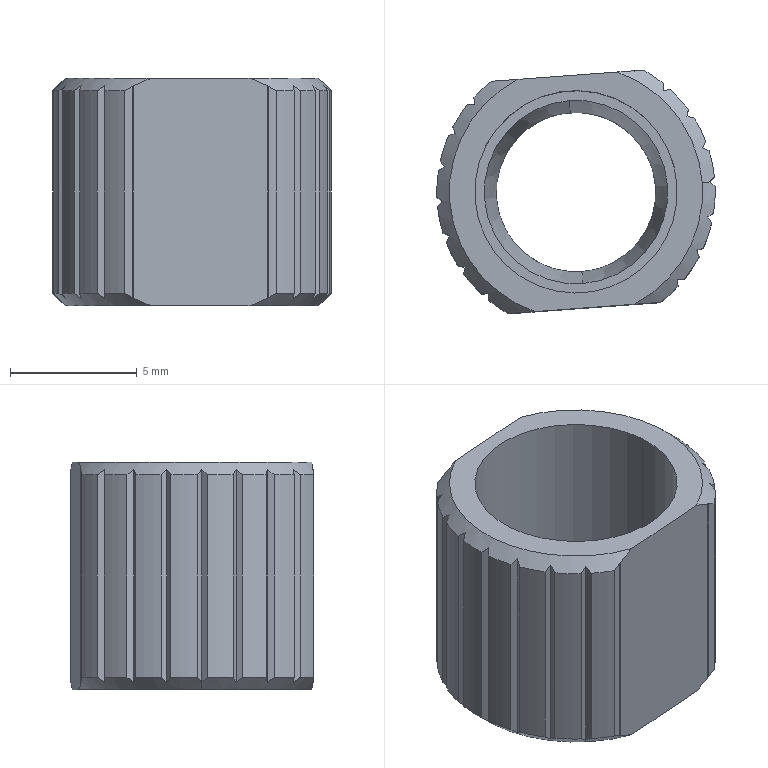Component | SolidWorks | MotorAssemblyWhen2-1_37bi-mpp70-3021-1 | 1 solid | 73 faces | volume 372 mm3 | plane 45 | cylinder 20 | cone 8 | commonest cylinder face diameters 11 x16 8 x2 6.3 x2